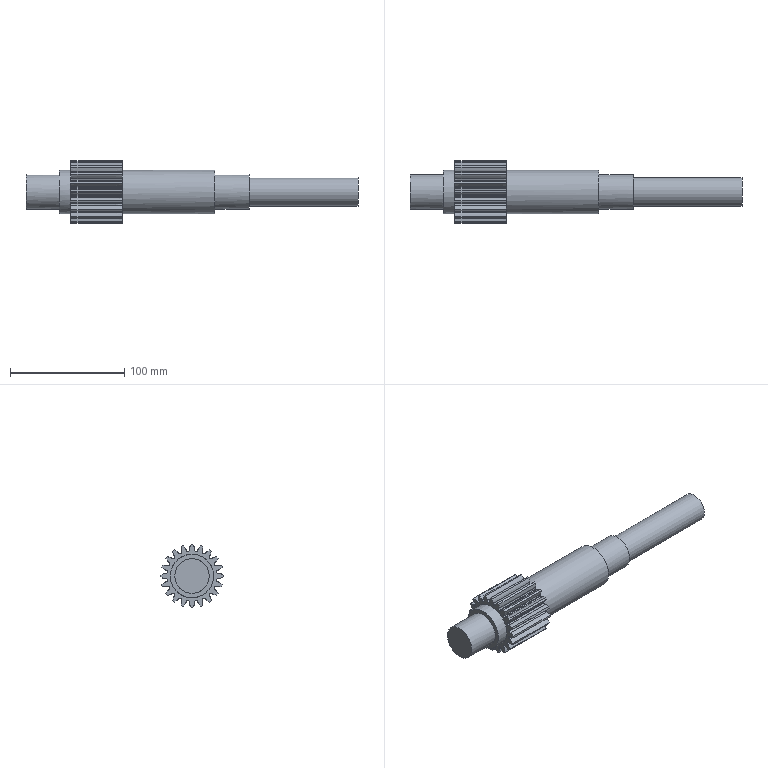Component | NX | SHURUZHOU | 1 solid | 132 faces | volume 278372 mm3 | other 100 | cylinder 25 | plane 7 | commonest cylinder face diameters 43.75 x20 38 x2 30 x2 25 x1